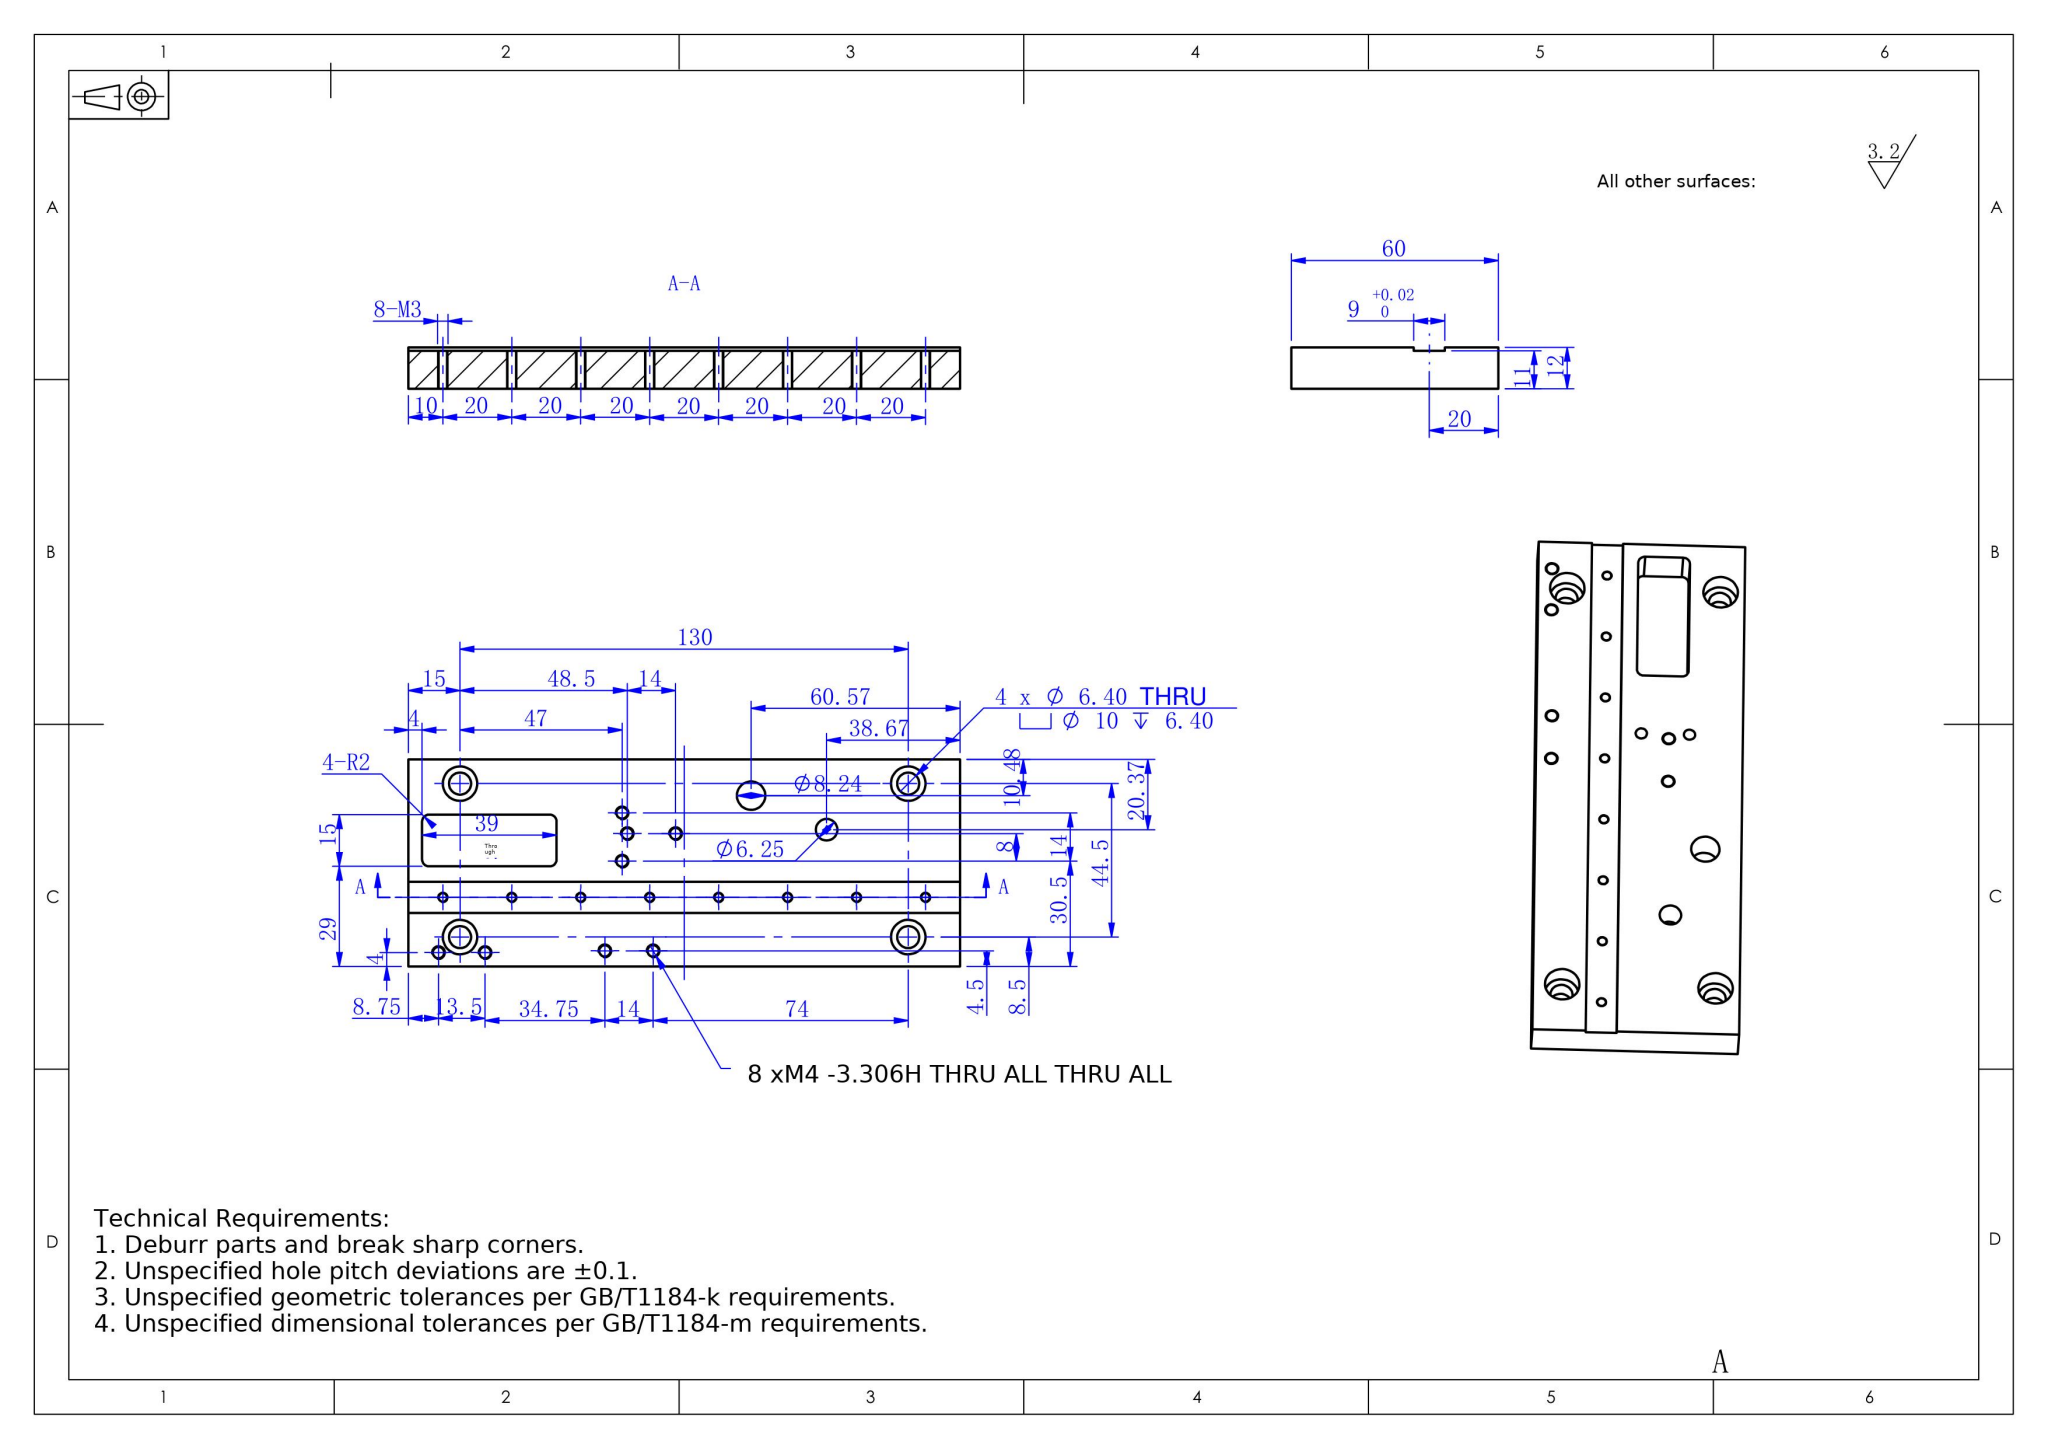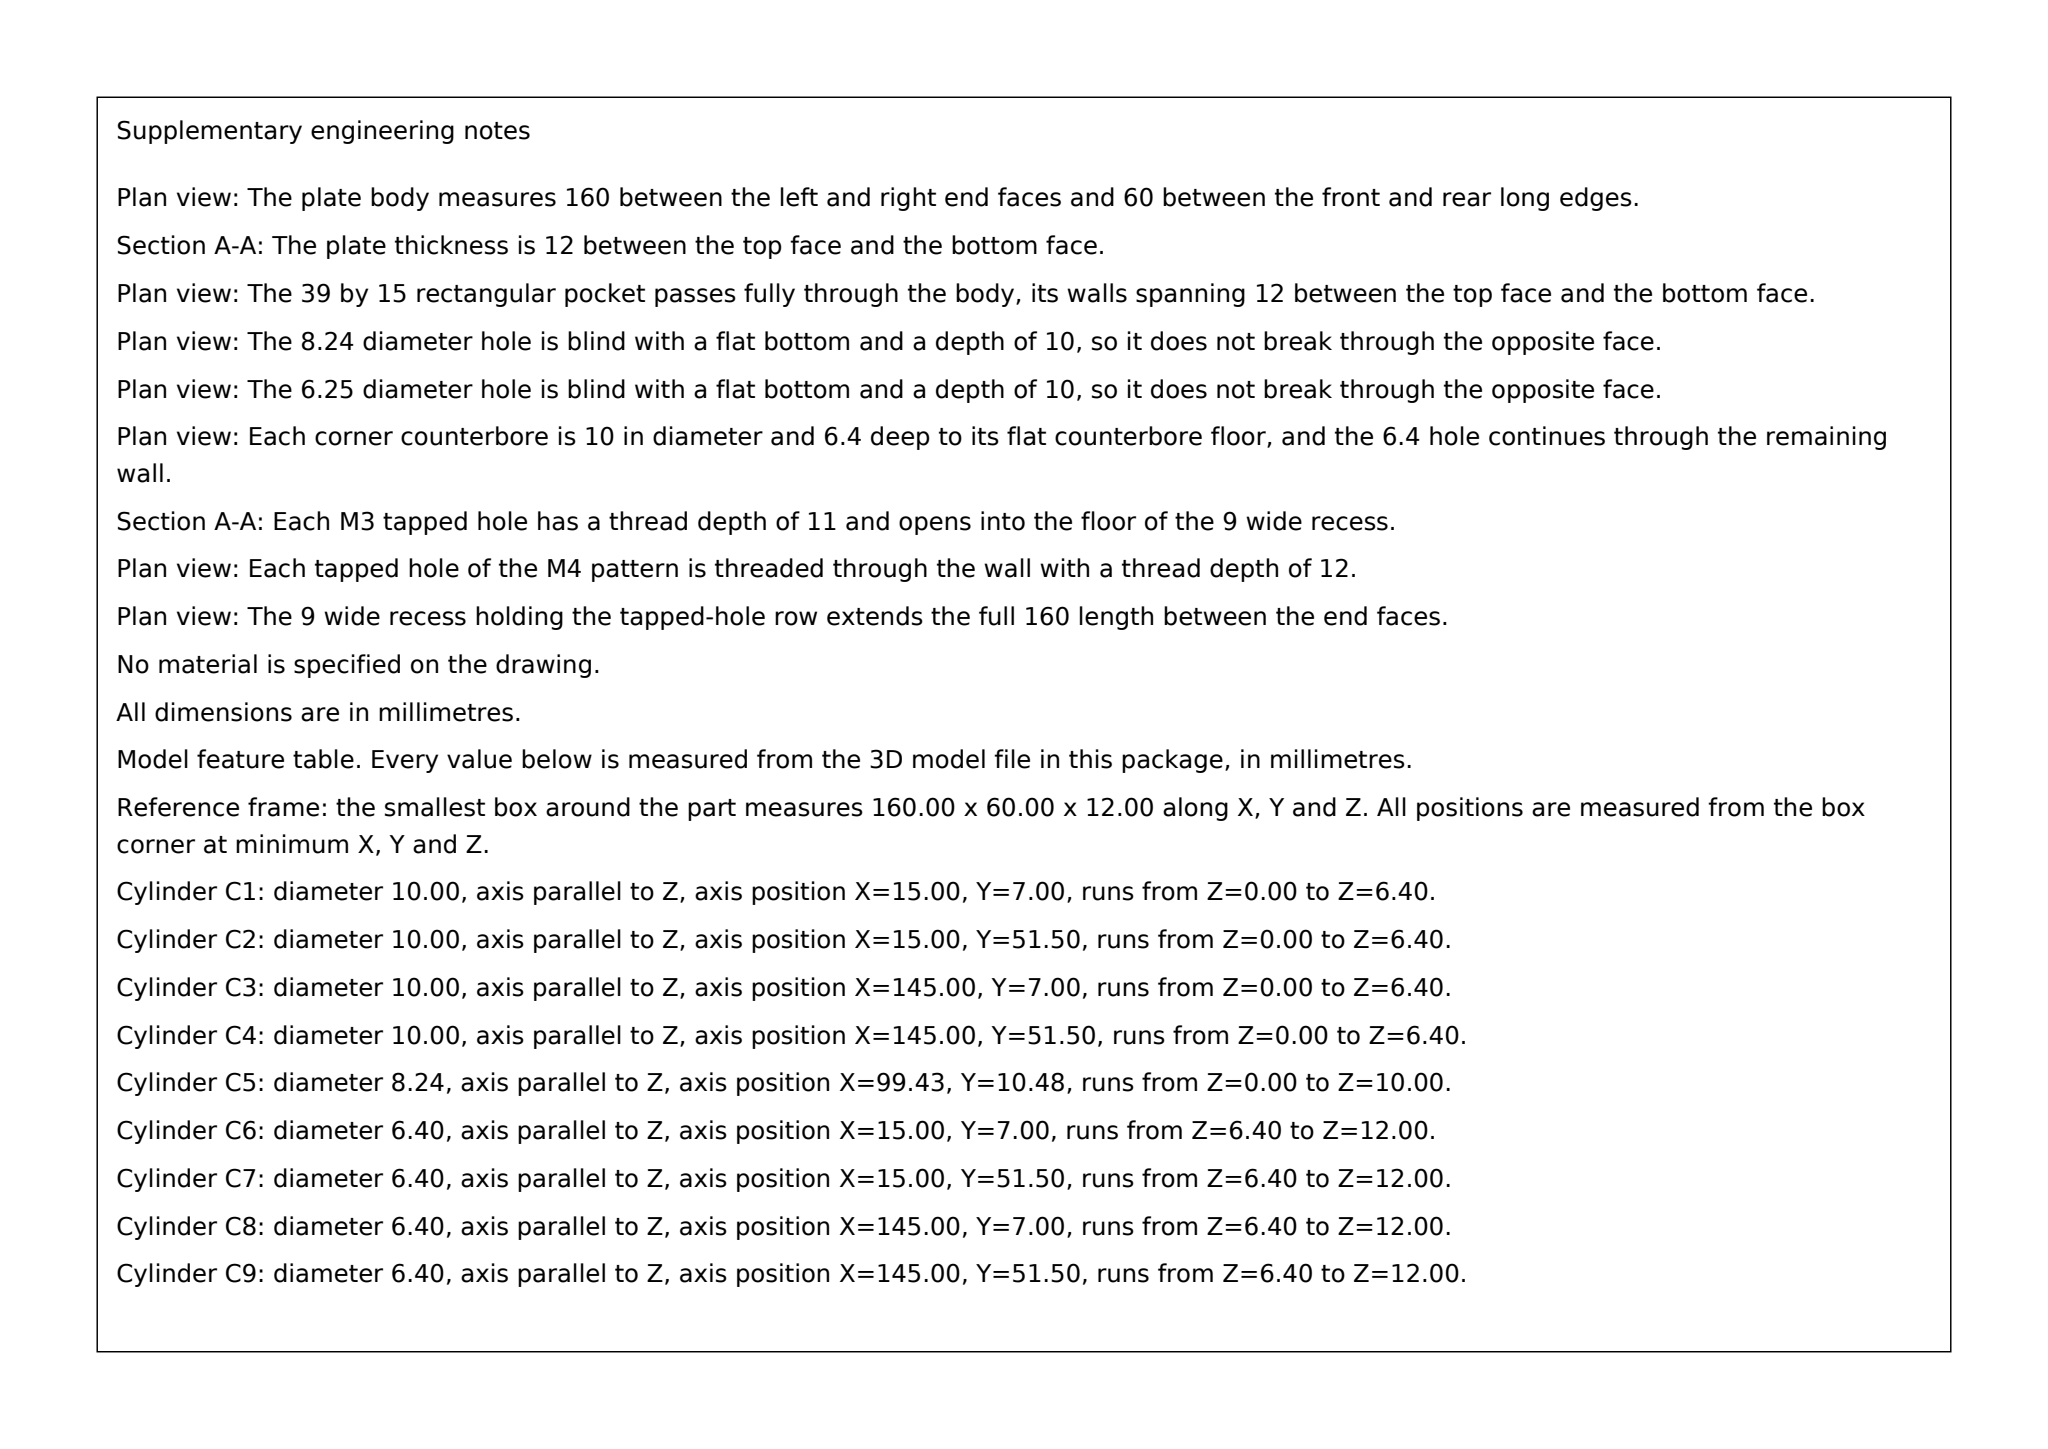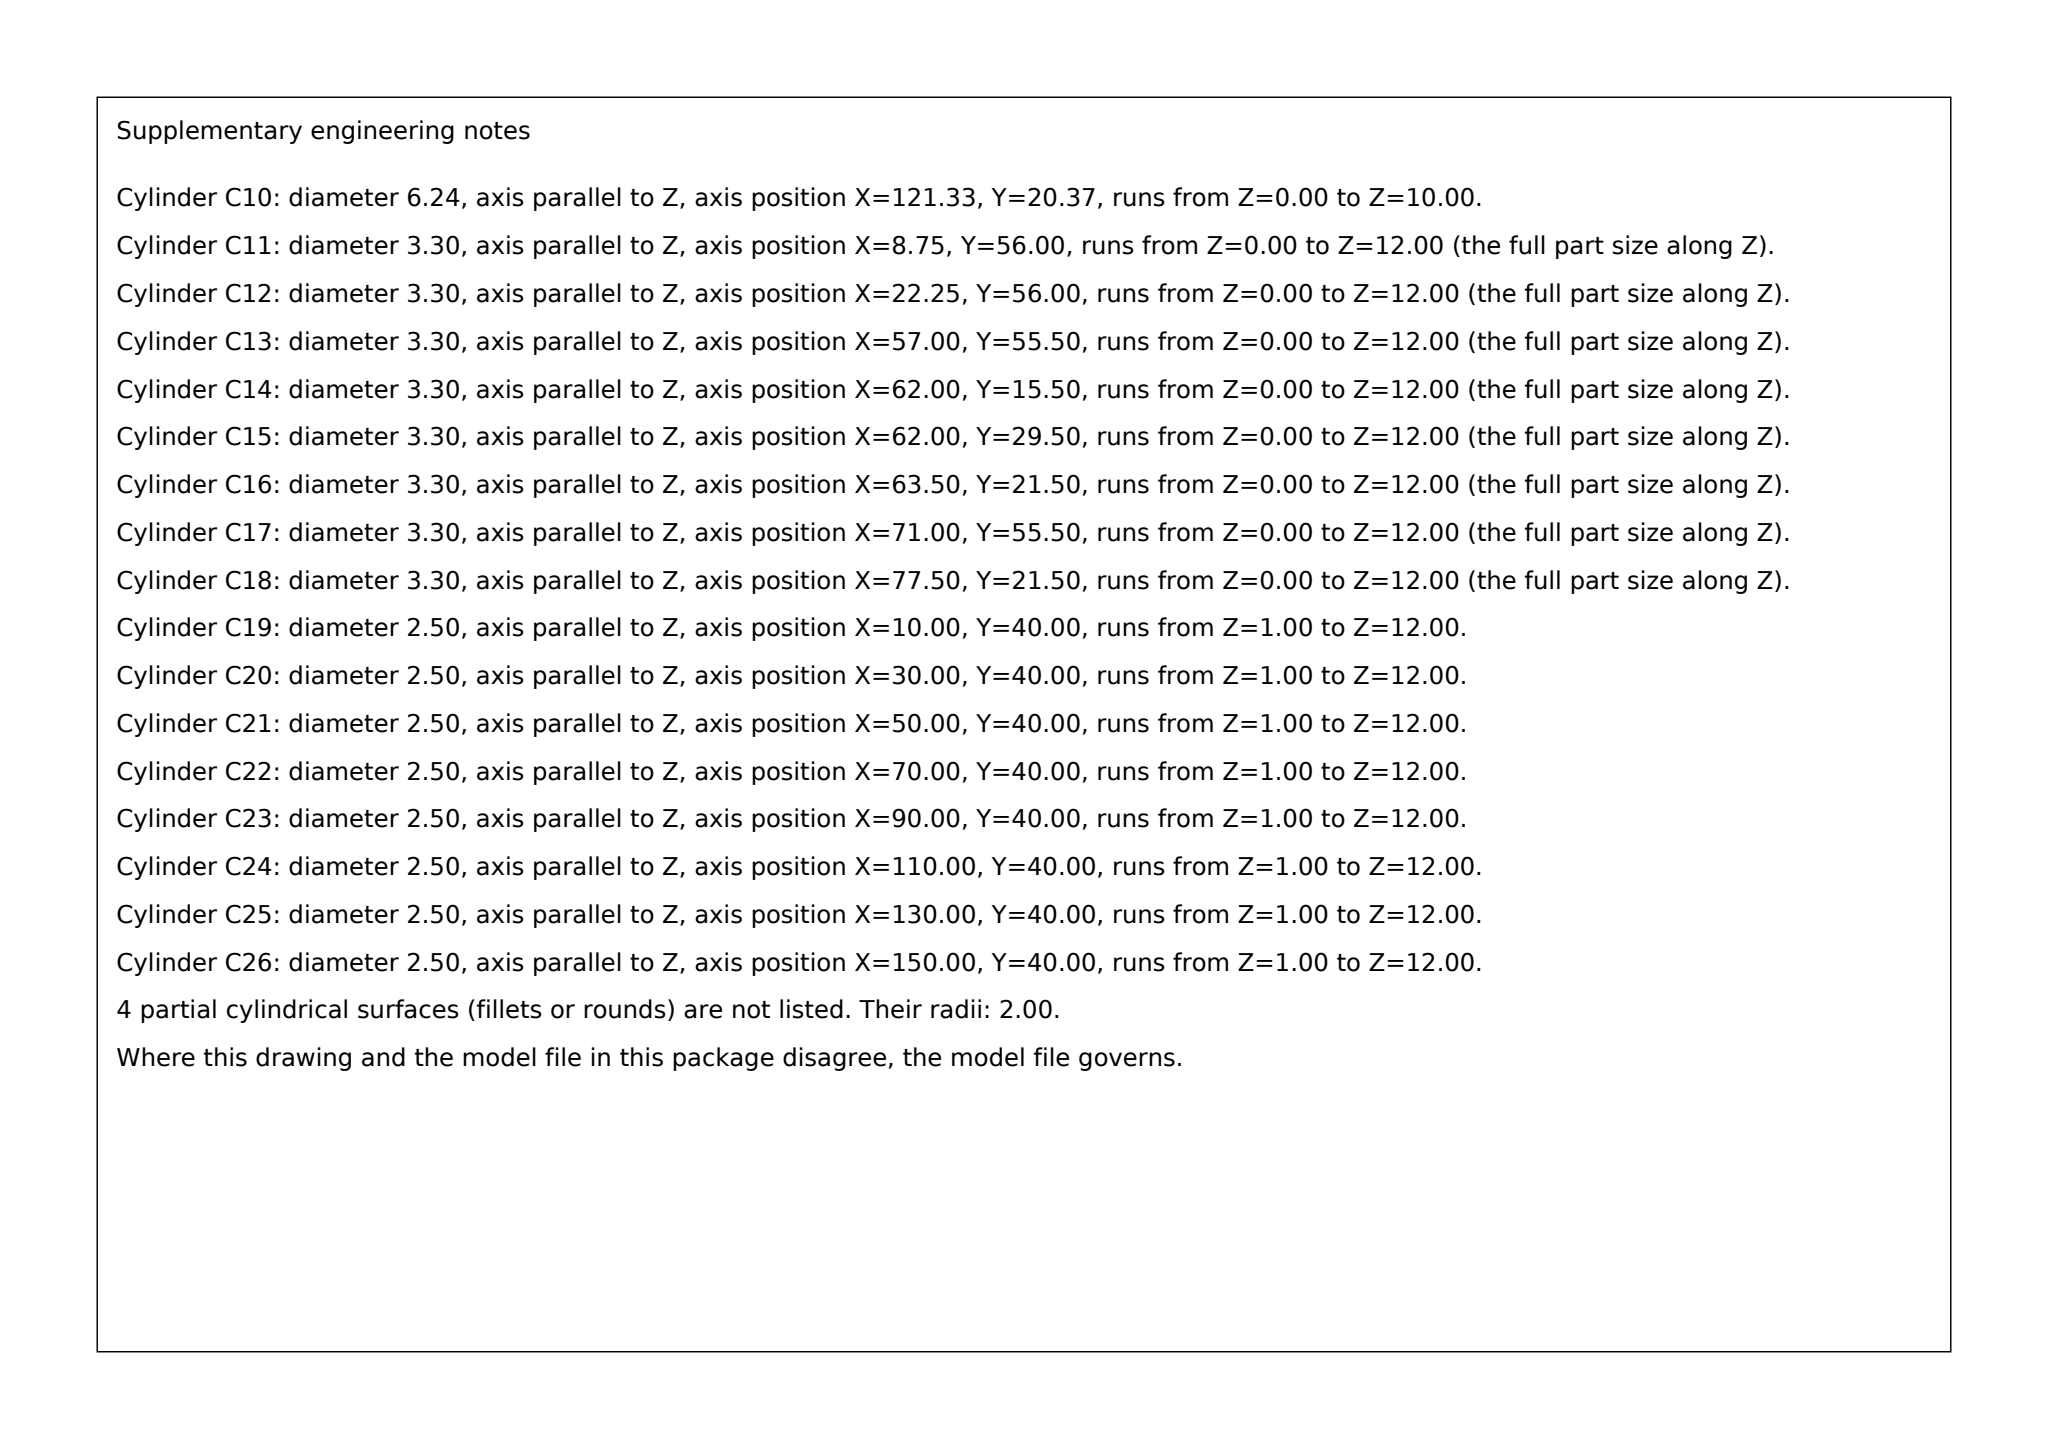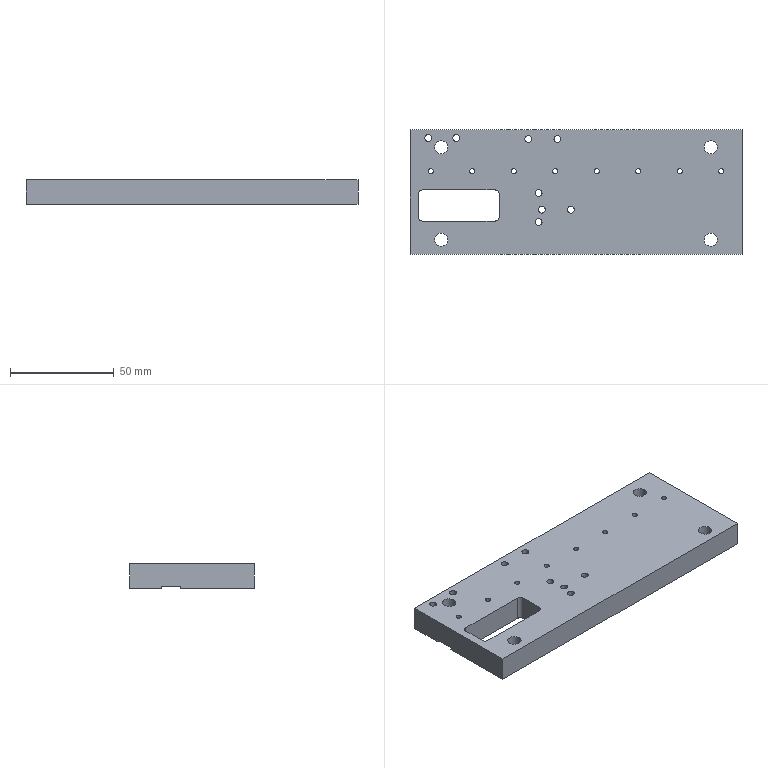Part | SolidWorks | mm | 1 solid | 76 faces | box 160 x 60 x 12 mm | volume 101957 mm3 | cylinder 56 | plane 20 | commonest cylinder face diameters 3.3 x16 2.5 x16 10 x8 6.4 x8 4 x4 6.249 x2 8.239 x2
Drawing notes:
4X Ø6.40 CBORE HOLES: UPPER PAIR 7 FROM TOP EDGE | from the solid: Ø6.4/Ø10 cbores at y=51.5 & 7.0 in 60 wide part: 60-51.5=8.5, 7.0 from opposite edge
build123d program:
from build123d import *

# Parameters (mm, degrees)
SKETCH1_W                                       = 160
SKETCH1_H                                       = 40
BOSS_EXTRUDE1_DEPTH                             = 12
SKETCH2_W                                       = 1
SKETCH2_H                                       = 9
CUT_EXTRUDE1_DEPTH                              = 169.751
SKETCH5_W                                       = 160
SKETCH5_H                                       = 12
BOSS_EXTRUDE2_DEPTH                             = 20
SKETCH6_W                                       = 39
SKETCH6_H                                       = 15
CUT_EXTRUDE2_DEPTH                              = 109.823
FILLET1_R                                       = 2
M4_TAPPED_HOLE1_D                               = 3.3
M4_TAPPED_HOLE2_D                               = 3.3
M4_TAPPED_HOLE3_D                               = 3.3
M3_TAPPED_HOLE2_D                               = 2.5
M4_TAPPED_HOLE5_D                               = 3.3
M6_HEX_SOCKET_HEAD_CAP_SCREW_CBORE2_D           = 6.4
M6_HEX_SOCKET_HEAD_CAP_SCREW_CBORE2_CBORE_D     = 10
M6_HEX_SOCKET_HEAD_CAP_SCREW_CBORE2_CBORE_DEPTH = 6.4
SKETCH27_R                                      = 3.125
SKETCH27_R_2                                    = 4.119
CUT_EXTRUDE3_DEPTH                              = 10


with BuildPart() as part:
    # Sketch1 → Boss-Extrude1 (new body)
    with BuildSketch(Plane.XY):
        with Locations((-14.686, 32.278)):
            Rectangle(SKETCH1_W, SKETCH1_H)
    extrude(amount=BOSS_EXTRUDE1_DEPTH)

    # Sketch2 → Cut-Extrude1 (cut, through all)
    with BuildSketch(Plane(origin=(65.314, 0, 0), x_dir=(0, 0, -1), z_dir=(1, 0, 0))):
        with Locations((-0.5, 32.278)):
            Rectangle(SKETCH2_W, SKETCH2_H)
    extrude(amount=-CUT_EXTRUDE1_DEPTH, mode=Mode.SUBTRACT)

    # Sketch5 → Boss-Extrude2 (add)
    with BuildSketch(Plane(origin=(0, 12.278, 0), x_dir=(-1, 0, 0), z_dir=(0, -1, 0))):
        with Locations((14.686, -6)):
            Rectangle(SKETCH5_W, SKETCH5_H)
    extrude(amount=BOSS_EXTRUDE2_DEPTH)

    # Sketch6 → Cut-Extrude2 (cut, through all)
    with BuildSketch(Plane(origin=(0, 0, 0), x_dir=(-1, 0, 0), z_dir=(0, 0, -1))):
        with Locations((71.186, 15.778)):
            Rectangle(SKETCH6_W, SKETCH6_H)
    extrude(amount=-CUT_EXTRUDE2_DEPTH, mode=Mode.SUBTRACT)

    # Fillet1
    fillet1_edges = [part.edges().sort_by_distance(p)[0] for p in [
        (-90.686, 23.278, 6),
        (-90.686, 8.278, 6),
        (-51.686, 8.278, 6),
        (-51.686, 23.278, 6),
    ]]
    fillet(fillet1_edges, radius=FILLET1_R)

    # M4 Tapped Hole1 (through all)
    with Locations(Plane.XY.offset(12)):
        with Locations((-32.686, 7.778), (-32.686, 21.778)):
            Hole(M4_TAPPED_HOLE1_D / 2)

    # M4 Tapped Hole2 (through all)
    with Locations(Plane(origin=(0, 0, 0), x_dir=(-1, 0, 0), z_dir=(0, 0, -1))):
        with Locations((85.936, 48.278), (72.436, 48.278)):
            Hole(M4_TAPPED_HOLE2_D / 2)

    # M4 Tapped Hole3 (through all)
    with Locations(Plane(origin=(0, 0, 0), x_dir=(-1, 0, 0), z_dir=(0, 0, -1))):
        with Locations((37.686, 47.778), (23.686, 47.778)):
            Hole(M4_TAPPED_HOLE3_D / 2)

    # M3 Tapped Hole2 (through all)
    with Locations(Plane(origin=(0, 0, 1), x_dir=(-1, 0, 0), z_dir=(0, 0, -1))):
        with Locations((84.686, 32.278), (64.686, 32.278), (44.686, 32.278), (24.686, 32.278), (4.686, 32.278), (-15.314, 32.278), (-35.314, 32.278), (-55.314, 32.278)):
            Hole(M3_TAPPED_HOLE2_D / 2)

    # M4 Tapped Hole5 (through all)
    with Locations(Plane(origin=(0, 0, 0), x_dir=(-1, 0, 0), z_dir=(0, 0, -1))):
        with Locations((17.186, 13.778), (31.186, 13.778)):
            Hole(M4_TAPPED_HOLE5_D / 2)

    # M6 Hex Socket Head Cap Screw CBORE2 (through all)
    with Locations(Plane(origin=(0, 0, 0), x_dir=(-1, 0, 0), z_dir=(0, 0, -1))):
        with Locations((-50.314, 43.778), (79.686, 43.778), (-50.314, -0.7223), (79.686, -0.7223)):
            CounterBoreHole(M6_HEX_SOCKET_HEAD_CAP_SCREW_CBORE2_D / 2, M6_HEX_SOCKET_HEAD_CAP_SCREW_CBORE2_CBORE_D / 2, M6_HEX_SOCKET_HEAD_CAP_SCREW_CBORE2_CBORE_DEPTH)

    # Sketch27 → Cut-Extrude3 (cut)
    with BuildSketch(Plane(origin=(0, 0, 0), x_dir=(-1, 0, 0), z_dir=(0, 0, -1))):
        with Locations((-26.642, 12.652)):
            Circle(SKETCH27_R)
        with Locations((-4.742, 2.762)):
            Circle(SKETCH27_R_2)
    extrude(amount=-CUT_EXTRUDE3_DEPTH, mode=Mode.SUBTRACT)


solid = part.part